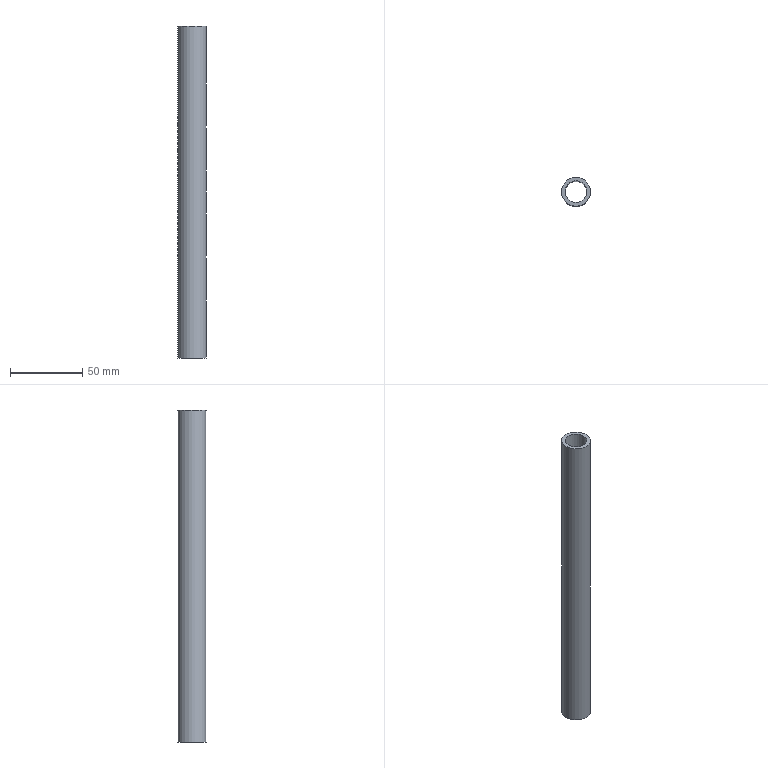Component | NX | SUPPORT_ROD_2 | 1 solid | 10 faces | volume 31315 mm3 | cylinder 8 | plane 2 | commonest cylinder face diameters 5 x6 20 x1 15 x1